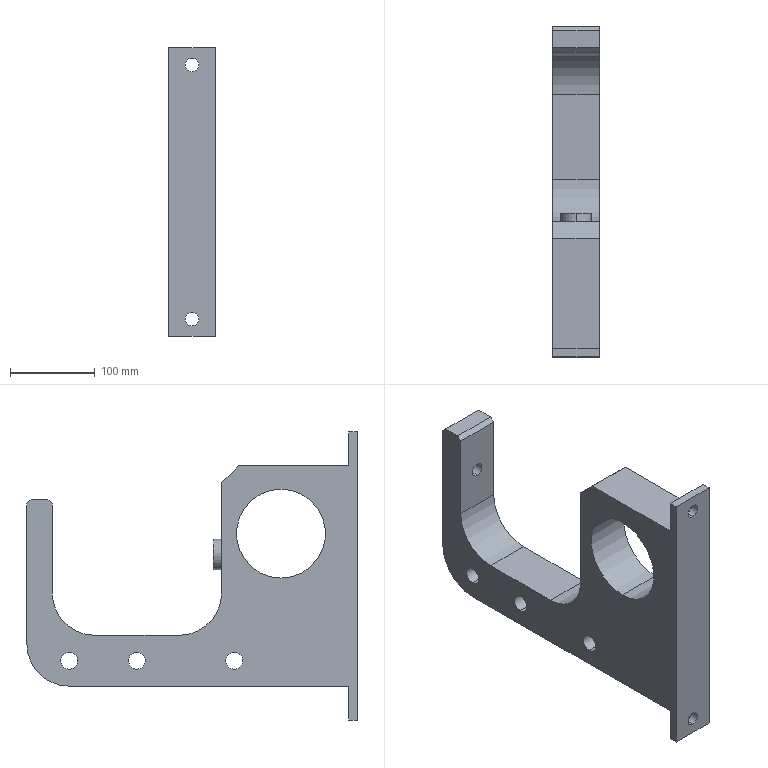Component | SolidWorks | dudukan-1 | 1 solid | 40 faces | box 55 x 390 x 340 mm | volume 2837108 mm3 | cylinder 21 | plane 19 | commonest cylinder face diameters 16 x6 20 x6 100 x3 30 x2 36 x2 105 x2 | material ASTM A36 Steel
build123d program:
from build123d import *

# Parameters (mm, degrees)
BOSS_EXTRUDE1_DEPTH      = 27.5
BOSS_EXTRUDE1_DEPTH_BACK = 27.5
SKETCH1_R                = 10
SKETCH1_R_2              = 52.5
SKETCH3_W                = 55
SKETCH3_H                = 340
BOSS_EXTRUDE3_DEPTH      = 10
SKETCH4_R                = 8
CUT_EXTRUDE1_DEPTH       = 422.374
CUT_EXTRUDE2_REACH       = 432.414
SKETCH5_R                = 8
SKETCH6_R                = 18
SKETCH6_R_2              = 15
BOSS_EXTRUDE4_DEPTH      = 10


with BuildPart() as part:
    # Sketch1 → Boss-Extrude1 (new, two sides: drawn at the far end of the back side and taken through both)
    with BuildSketch(Plane(origin=(0, 0, 0), x_dir=(0, 0, -1), z_dir=(1, 0, 0)).offset(-BOSS_EXTRUDE1_DEPTH_BACK)):
        with BuildLine():
            ThreePointArc((30, -40), (65.355, -25.355), (80, 10))
            Line((80, 10), (80, 110))
            ThreePointArc((80, 110), (65.355, 145.355), (30, 160))
            Line((30, 160), (-75, 160))
            Line((-75, 160), (-80, 165))
            Line((-80, 165), (-80, 185))
            Line((-80, 185), (-75, 190))
            Line((-75, 190), (90, 190))
            ThreePointArc((90, 190), (125.355, 175.355), (140, 140))
            Line((140, 140), (140, -190))
            Line((140, -190), (-120, -190))
            Line((-120, -190), (-120, -60))
            Line((-120, -60), (-100, -40))
            Line((-100, -40), (30, -40))
        make_face()
        with Locations((110, 60)):
            Circle(SKETCH1_R, mode=Mode.SUBTRACT)
        with Locations((110, -55)):
            Circle(SKETCH1_R, mode=Mode.SUBTRACT)
        with Locations((110, 140)):
            Circle(SKETCH1_R, mode=Mode.SUBTRACT)
        with Locations((-40, -110)):
            Circle(SKETCH1_R_2, mode=Mode.SUBTRACT)
    extrude(amount=BOSS_EXTRUDE1_DEPTH + BOSS_EXTRUDE1_DEPTH_BACK)

    # Sketch3 → Boss-Extrude3 (add)
    with BuildSketch(Plane.XZ.offset(190)):
        with Locations((0, -10)):
            Rectangle(SKETCH3_W, SKETCH3_H)
    extrude(amount=BOSS_EXTRUDE3_DEPTH)

    # Sketch4 → Cut-Extrude1 (cut, through all)
    with BuildSketch(Plane(origin=(0, -190, 0), x_dir=(1, 0, 0), z_dir=(0, 1, 0))):
        with Locations(Location((0, 160, 0), (0, 0, 270))):
            Circle(SKETCH4_R)
        with Locations(Location((0, -140, 0), (0, 0, 270))):
            Circle(SKETCH4_R)
    extrude(amount=-CUT_EXTRUDE1_DEPTH, mode=Mode.SUBTRACT)

    # Sketch5 → Cut-Extrude2 (cut, up to next)
    with BuildSketch(Plane(origin=(0, 190, 0), x_dir=(1, 0, 0), z_dir=(0, 1, 0)), mode=Mode.PRIVATE) as cut_extrude2_sk1:
        with Locations(Location((0, -20, 0), (0, 0, 270))):
            Circle(SKETCH5_R)
    cut_extrude2_tool1 = extrude(cut_extrude2_sk1.sketch, amount=-CUT_EXTRUDE2_REACH, mode=Mode.PRIVATE) & part.part
    add(cut_extrude2_tool1.solids().sort_by_distance((0, 190, 20))[0], mode=Mode.SUBTRACT)

    # Sketch6 → Boss-Extrude4 (add)
    with BuildSketch(Plane(origin=(0, -40, 0), x_dir=(1, 0, 0), z_dir=(0, 1, 0))):
        with Locations(Location((0, -15.416, 0), (0, 0, 90))):
            Circle(SKETCH6_R)
        with Locations(Location((0, -15.416, 0), (0, 0, 90))):
            Circle(SKETCH6_R_2, mode=Mode.SUBTRACT)
    extrude(amount=BOSS_EXTRUDE4_DEPTH)


solid = part.part